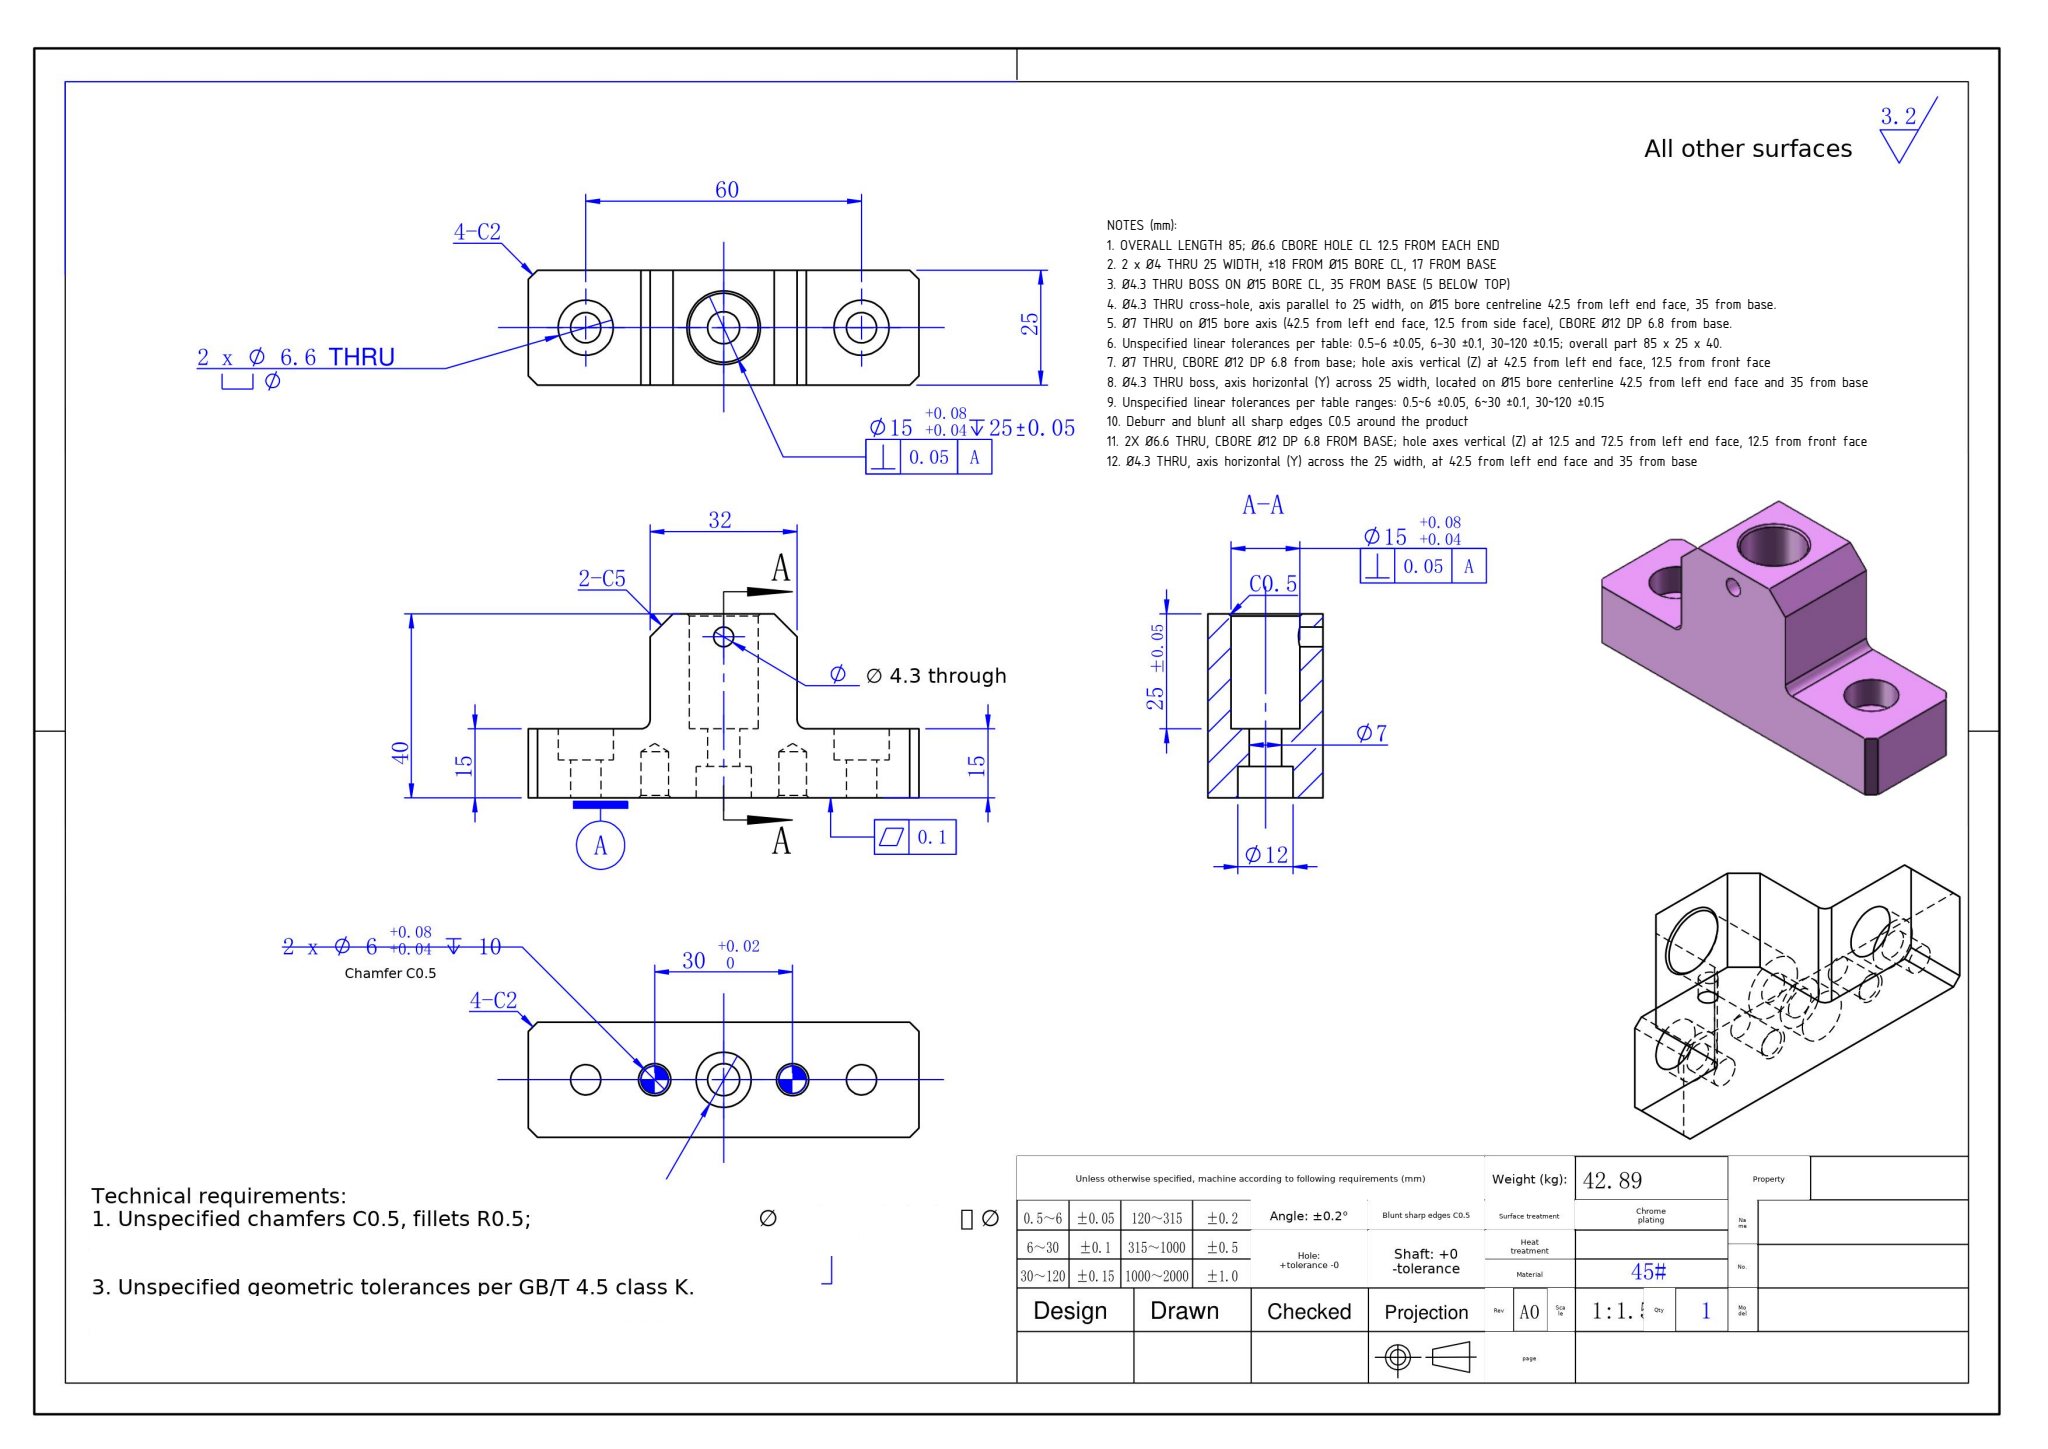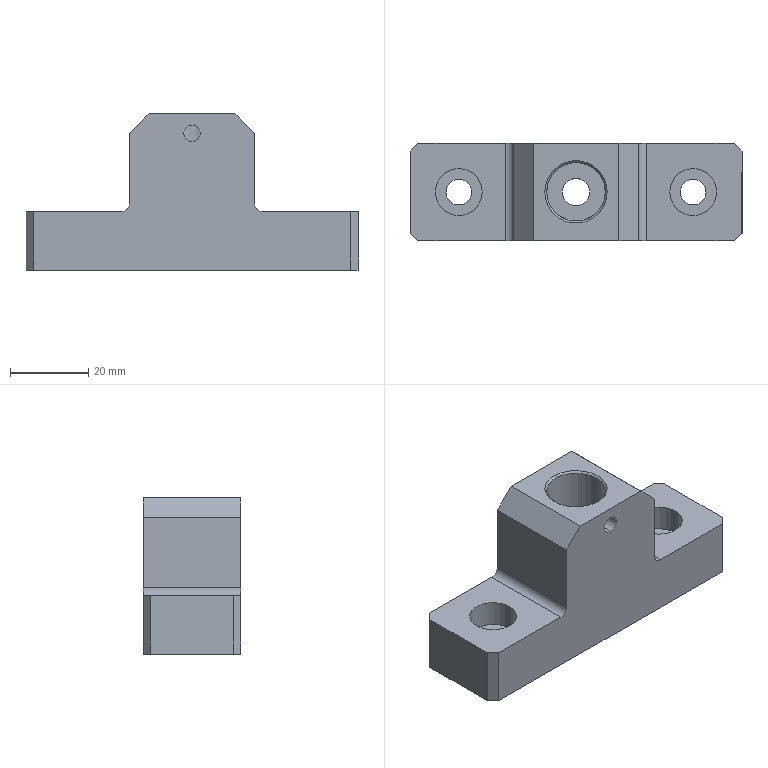Part | SolidWorks | mm | 1 solid | 52 faces | box 85 x 25 x 40 mm | volume 42887 mm3 | cylinder 22 | plane 20 | cone 10 | commonest cylinder face diameters 12 x6 6 x4 6.6 x4 4.3 x2 7 x2 15 x2 4 x2
Drawing notes:
OVERALL LENGTH 85; Ø6.6 CBORE HOLE CL 12.5 FROM EACH END | from the solid: bbox_xyz x=85.0; Ø6.6 cyl at x=12.5 and x=72.5 (85-72.5=12.5)
2 x Ø4 THRU 25 WIDTH, ±18 FROM Ø15 BORE CL, 17 FROM BASE | from the solid: cyls [4.0,'y',[24.5,-,17.0],25.0] & [4.0,'y',[60.5,-,17.0],25.0]; 42.5-24.5=18, 60.5-42.5=18; z=17 from z=0; len 25 = full Y
Ø4.3 THRU BOSS ON Ø15 BORE CL, 35 FROM BASE (5 BELOW TOP) | from the solid: Ø4.3 axis y at x=42.5 (=Ø15 bore CL), z=35.0; top face z=40.0, base z=0
Ø4.3 THRU cross-hole, axis parallel to 25 width, on Ø15 bore centreline 42.5 from left end face, 35 from base. | from the solid: cylinders: [4.3,"y",[42.5,null,35.0],5.32]
Ø7 THRU on Ø15 bore axis (42.5 from left end face, 12.5 from side face), CBORE Ø12 DP 6.8 from base. | from the solid: cylinders: [7.0,"z",[42.5,12.5,null],8.2] and [12.0,"z",[42.5,12.5,null],6.8]
Unspecified linear tolerances per table: 0.5-6 ±0.05, 6-30 ±0.1, 30-120 ±0.15; overall part 85 x 25 x 40. | from the solid: bbox_xyz [85.0,25.0,40.0]
Ø7 THRU, CBORE Ø12 DP 6.8 from base; hole axis vertical (Z) at 42.5 from left end face, 12.5 from front face | from the solid: cylinders: [7.0,'z',[42.5,12.5],8.2] and [12.0,'z',[42.5,12.5],6.8]; bbox_xyz 85x25x40
Ø4.3 THRU boss, axis horizontal (Y) across 25 width, located on Ø15 bore centerline 42.5 from left end face and 35 from base | from the solid: cylinders: [4.3,'y',[42.5,null,35.0],5.32]
Unspecified linear tolerances per table ranges: 0.5~6 ±0.05, 6~30 ±0.1, 30~120 ±0.15 | from the solid: title-block tolerance table (sheet) consistent with bbox_xyz 85x25x40 feature sizes
Deburr and blunt all sharp edges C0.5 around the product | from the solid: cones[90.0,6.0] chamfer cones and axis_planes z 8.2/15.0 edges
2X Ø6.6 THRU, CBORE Ø12 DP 6.8 FROM BASE; hole axes vertical (Z) at 12.5 and 72.5 from left end face, 12.5 from front face | from the solid: cylinders: [6.6,z,(12.5,12.5),8.2] and [6.6,z,(72.5,12.5),8.2]; [12.0,z,(12.5,12.5),6.8] and [12.0,z,(72.5,12.5),6.8]; bbox 85 x 25 x 40
Ø4.3 THRU, axis horizontal (Y) across the 25 width, at 42.5 from left end face and 35 from base | from the solid: cylinder [4.3,y,(42.5,null,35.0),5.32]; axis plane y=0 and y=25
build123d program:
from build123d import *

# Parameters (mm, degrees)
SKETCH1_W                                         = 85
SKETCH1_H                                         = 25
BOSS_EXTRUDE1_DEPTH                               = 20
SKETCH2_R                                         = 7.5
CUT_EXTRUDE1_DEPTH                                = 25
HOLE_SIZE_ACCORDING_TO_HEXAGON_SOCKET_D           = 7
HOLE_SIZE_ACCORDING_TO_HEXAGON_SOCKET_CBORE_D     = 12
HOLE_SIZE_ACCORDING_TO_HEXAGON_SOCKET_CBORE_DEPTH = 6.8
CHAMFER1_SIZE                                     = 2
CHAMFER2_SIZE                                     = 0.5
SKETCH5_W                                         = 26.5
SKETCH5_H                                         = 25
CUT_EXTRUDE2_DEPTH                                = 25
HOLE_SIZE_ACCORDING_TO_HEXAGON_SO_2_D             = 6.6
HOLE_SIZE_ACCORDING_TO_HEXAGON_SO_2_CBORE_D       = 12
HOLE_SIZE_ACCORDING_TO_HEXAGON_SO_2_CBORE_DEPTH   = 6.8
CHAMFER3_SIZE                                     = 5
M4_CLEARANCE_HOLE_1_REACH                         = 55.209
M4_CLEARANCE_HOLE_1_BORE_R                        = 2.15
SIZE_MM_DOWEL_PIN_HOLE_1_D                        = 6
SIZE_MM_DOWEL_PIN_HOLE_1_DEPTH                    = 10
SIZE_MM_DOWEL_PIN_HOLE_1_TIP                      = 1.803
CHAMFER4_SIZE                                     = 0.5
FILLET1_R                                         = 2


with BuildPart() as part:
    # Sketch1 → Boss-Extrude1 (new, symmetric)
    with BuildSketch(Plane.XY):
        Rectangle(SKETCH1_W, SKETCH1_H)
    extrude(amount=BOSS_EXTRUDE1_DEPTH, both=True)

    # Sketch2 → Cut-Extrude1 (cut)
    with BuildSketch(Plane.XY.offset(20)):
        Circle(SKETCH2_R)
    extrude(amount=-CUT_EXTRUDE1_DEPTH, mode=Mode.SUBTRACT)

    # Hole Size _ according to_ Hexagon Socket (through all)
    with Locations(Plane(origin=(0, 0, -20), x_dir=(-1, 0, 0), z_dir=(0, 0, -1))):
        with Locations((0, 0)):
            CounterBoreHole(HOLE_SIZE_ACCORDING_TO_HEXAGON_SOCKET_D / 2, HOLE_SIZE_ACCORDING_TO_HEXAGON_SOCKET_CBORE_D / 2, HOLE_SIZE_ACCORDING_TO_HEXAGON_SOCKET_CBORE_DEPTH)

    # Chamfer1
    chamfer1_edges = [part.edges().sort_by_distance(p)[0] for p in [
        (-42.5, 12.5, 0),
        (42.5, 12.5, 0),
        (42.5, -12.5, 0),
        (-42.5, -12.5, 0),
    ]]
    chamfer(chamfer1_edges, length=CHAMFER1_SIZE)

    # Chamfer2
    chamfer2_edges = [part.edges().sort_by_distance(p)[0] for p in [
        (-7.5, 0, 20),
    ]]
    chamfer(chamfer2_edges, length=CHAMFER2_SIZE)

    # Sketch5 → Cut-Extrude2 (cut)
    with BuildSketch(Plane.XY.offset(20)):
        with Locations((-29.25, 0)):
            Rectangle(SKETCH5_W, SKETCH5_H)
    cut_extrude2 = extrude(amount=-CUT_EXTRUDE2_DEPTH, mode=Mode.SUBTRACT)

    # Mirror1: Cut-Extrude2 across plane
    add(cut_extrude2.mirror(Plane(origin=(0, 0, 0), x_dir=(0, 0, 1), z_dir=(1, 0, 0))), mode=Mode.SUBTRACT)

    # Hole Size _ according to_ Hexagon So 2 (through all)
    with Locations(Plane.XY.offset(-5)):
        with Locations((-30, 0), (30, 0)):
            CounterBoreHole(HOLE_SIZE_ACCORDING_TO_HEXAGON_SO_2_D / 2, HOLE_SIZE_ACCORDING_TO_HEXAGON_SO_2_CBORE_D / 2, HOLE_SIZE_ACCORDING_TO_HEXAGON_SO_2_CBORE_DEPTH)

    # Chamfer3
    chamfer3_edges = [part.edges().sort_by_distance(p)[0] for p in [
        (-16, 0, 20),
        (16, 0, 20),
    ]]
    chamfer(chamfer3_edges, length=CHAMFER3_SIZE)

    # M4 Clearance Hole 1 bore → M4 Clearance Hole 1 (cut, up to next)
    with BuildSketch(Plane(origin=(0, -12.5, 0), x_dir=(-1, 0, 0), z_dir=(0, -1, 0)), mode=Mode.PRIVATE) as m4_clearance_hole_1_sk1:
        with Locations((0, -15)):
            Circle(M4_CLEARANCE_HOLE_1_BORE_R)
    m4_clearance_hole_1_tool1 = extrude(m4_clearance_hole_1_sk1.sketch, amount=-M4_CLEARANCE_HOLE_1_REACH, mode=Mode.PRIVATE) & part.part
    add(m4_clearance_hole_1_tool1.solids().sort_by_distance((0, -12.5, 15))[0], mode=Mode.SUBTRACT)

    # Size mm Dowel Pin Hole 1
    with Locations(Plane(origin=(0, 0, -20), x_dir=(-1, 0, 0), z_dir=(0, 0, -1))):
        with Locations((-15, 0), (15, 0)):
            Hole(SIZE_MM_DOWEL_PIN_HOLE_1_D / 2, depth=SIZE_MM_DOWEL_PIN_HOLE_1_DEPTH)
            with Locations((0, 0, -(SIZE_MM_DOWEL_PIN_HOLE_1_DEPTH + SIZE_MM_DOWEL_PIN_HOLE_1_TIP / 2))):  # 118° drill point
                Cone(0, SIZE_MM_DOWEL_PIN_HOLE_1_D / 2, SIZE_MM_DOWEL_PIN_HOLE_1_TIP, mode=Mode.SUBTRACT)

    # Chamfer4
    chamfer4_edges = [part.edges().sort_by_distance(p)[0] for p in [
        (-18, 0, -20),
        (12, 0, -20),
    ]]
    chamfer(chamfer4_edges, length=CHAMFER4_SIZE)

    # Fillet1
    fillet1_edges = [part.edges().sort_by_distance(p)[0] for p in [
        (-16, 0, -5),
        (16, 0, -5),
    ]]
    fillet(fillet1_edges, radius=FILLET1_R)


solid = part.part